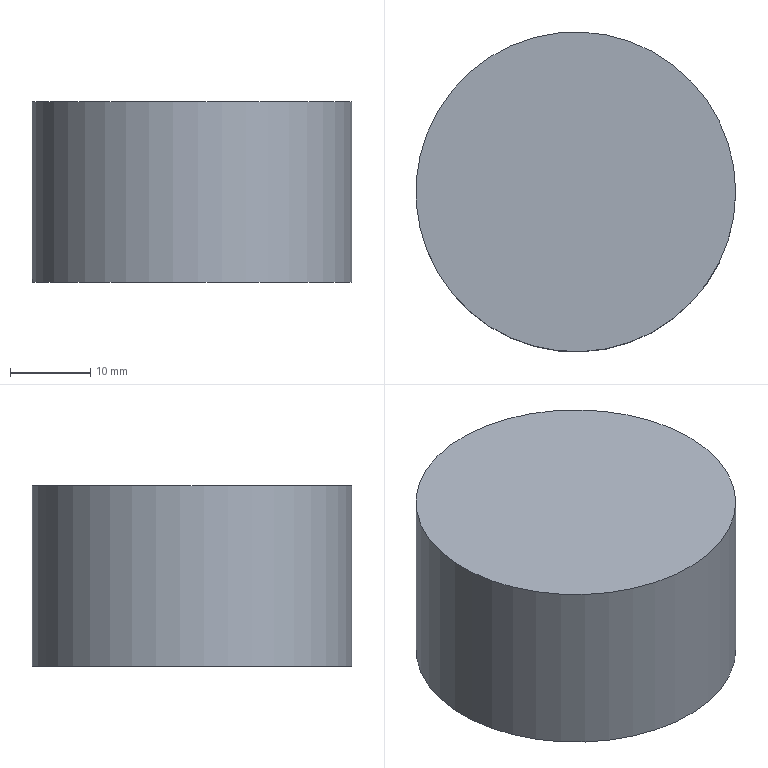Component | NX | SPEAKER | 1 solid | 3 faces | box 39.8 x 39.8 x 22.5 mm | volume 27992 mm3 | plane 2 | cylinder 1 | commonest cylinder face diameters 39.8 x1
STEP:
#1=CARTESIAN_POINT('',(0.,0.,0.));
#2=DIRECTION('',(0.,0.,1.));
#3=DIRECTION('',(1.,0.,0.));
#4=AXIS2_PLACEMENT_3D('',#1,#2,#3);
#5=CARTESIAN_POINT('',(62.178,-1.116,28.276));
#6=VERTEX_POINT('',#5);
#7=CARTESIAN_POINT('',(42.278,-1.116,28.276));
#8=DIRECTION('',(0.,0.,-1.));
#9=DIRECTION('',(1.,0.,0.));
#10=AXIS2_PLACEMENT_3D('',#7,#8,#9);
#11=CIRCLE('',#10,19.9);
#12=CARTESIAN_POINT('',(42.278,-1.116,28.276));
#13=DIRECTION('',(0.,0.,1.));
#14=DIRECTION('',(1.,0.,0.));
#15=AXIS2_PLACEMENT_3D('',#12,#13,#14);
#16=PLANE('',#15);
#17=CARTESIAN_POINT('',(19.9,0.));
#18=CARTESIAN_POINT('',(19.9,-34.468));
#19=CARTESIAN_POINT('',(-9.95,-17.234));
#20=CARTESIAN_POINT('',(-39.8,-0.));
#21=CARTESIAN_POINT('',(-9.95,17.234));
#22=CARTESIAN_POINT('',(19.9,34.468));
#23=CARTESIAN_POINT('',(19.9,0.));
#24=(BOUNDED_CURVE()B_SPLINE_CURVE(2,(#17,#18,#19,#20,#21,#22,#23),.UNSPECIFIED.,.T.,.F.)B_SPLINE_CURVE_WITH_KNOTS((1,2,2,2,2,1),(-2.094,0.,2.094,4.189,6.283,8.378),.UNSPECIFIED.)CURVE()GEOMETRIC_REPRESENTATION_ITEM()RATIONAL_B_SPLINE_CURVE((1.,0.5,1.,0.5,1.,0.5,1.))REPRESENTATION_ITEM(''));
#25=(GEOMETRIC_REPRESENTATION_CONTEXT(2)PARAMETRIC_REPRESENTATION_CONTEXT()REPRESENTATION_CONTEXT('',''));
#26=DEFINITIONAL_REPRESENTATION('',(#24),#25);
#27=PCURVE('',#16,#26);
#28=CARTESIAN_POINT('',(42.278,-1.116,5.776));
#29=DIRECTION('',(0.,0.,1.));
#30=DIRECTION('',(1.,0.,0.));
#31=AXIS2_PLACEMENT_3D('',#28,#29,#30);
#32=CYLINDRICAL_SURFACE('',#31,19.9);
#33=CARTESIAN_POINT('',(6.283,22.5));
#34=DIRECTION('',(-1.,0.));
#35=VECTOR('',#34,1.);
#36=LINE('',#33,#35);
#37=(GEOMETRIC_REPRESENTATION_CONTEXT(2)PARAMETRIC_REPRESENTATION_CONTEXT()REPRESENTATION_CONTEXT('',''));
#38=DEFINITIONAL_REPRESENTATION('',(#36),#37);
#39=PCURVE('',#32,#38);
#40=SURFACE_CURVE('',#11,(#27,#39),.PCURVE_S1.);
#41=EDGE_CURVE('',#6,#6,#40,.T.);
#42=ORIENTED_EDGE('',*,*,#41,.F.);
#43=EDGE_LOOP('',(#42));
#44=FACE_BOUND('',#43,.T.);
#45=ADVANCED_FACE('',(#44),#16,.T.);
#46=CARTESIAN_POINT('',(62.178,-1.116,5.776));
#47=VERTEX_POINT('',#46);
#48=CARTESIAN_POINT('',(42.278,-1.116,5.776));
#49=DIRECTION('',(0.,0.,1.));
#50=DIRECTION('',(1.,0.,0.));
#51=AXIS2_PLACEMENT_3D('',#48,#49,#50);
#52=CIRCLE('',#51,19.9);
#53=CARTESIAN_POINT('',(42.278,-1.116,5.776));
#54=DIRECTION('',(0.,0.,-1.));
#55=DIRECTION('',(-1.,0.,0.));
#56=AXIS2_PLACEMENT_3D('',#53,#54,#55);
#57=PLANE('',#56);
#58=CARTESIAN_POINT('',(-19.9,0.));
#59=CARTESIAN_POINT('',(-19.9,34.468));
#60=CARTESIAN_POINT('',(9.95,17.234));
#61=CARTESIAN_POINT('',(39.8,0.));
#62=CARTESIAN_POINT('',(9.95,-17.234));
#63=CARTESIAN_POINT('',(-19.9,-34.468));
#64=CARTESIAN_POINT('',(-19.9,0.));
#65=(BOUNDED_CURVE()B_SPLINE_CURVE(2,(#58,#59,#60,#61,#62,#63,#64),.UNSPECIFIED.,.T.,.F.)B_SPLINE_CURVE_WITH_KNOTS((1,2,2,2,2,1),(-2.094,0.,2.094,4.189,6.283,8.378),.UNSPECIFIED.)CURVE()GEOMETRIC_REPRESENTATION_ITEM()RATIONAL_B_SPLINE_CURVE((1.,0.5,1.,0.5,1.,0.5,1.))REPRESENTATION_ITEM(''));
#66=(GEOMETRIC_REPRESENTATION_CONTEXT(2)PARAMETRIC_REPRESENTATION_CONTEXT()REPRESENTATION_CONTEXT('',''));
#67=DEFINITIONAL_REPRESENTATION('',(#65),#66);
#68=PCURVE('',#57,#67);
#69=CARTESIAN_POINT('',(0.,0.));
#70=DIRECTION('',(1.,0.));
#71=VECTOR('',#70,1.);
#72=LINE('',#69,#71);
#73=(GEOMETRIC_REPRESENTATION_CONTEXT(2)PARAMETRIC_REPRESENTATION_CONTEXT()REPRESENTATION_CONTEXT('',''));
#74=DEFINITIONAL_REPRESENTATION('',(#72),#73);
#75=PCURVE('',#32,#74);
#76=SURFACE_CURVE('',#52,(#68,#75),.PCURVE_S1.);
#77=EDGE_CURVE('',#47,#47,#76,.T.);
#78=ORIENTED_EDGE('',*,*,#77,.F.);
#79=EDGE_LOOP('',(#78));
#80=FACE_BOUND('',#79,.T.);
#81=ADVANCED_FACE('',(#80),#57,.T.);
#82=ORIENTED_EDGE('',*,*,#41,.T.);
#83=CARTESIAN_POINT('',(62.178,-1.116,5.776));
#84=CARTESIAN_POINT('',(62.178,-1.116,28.276));
#85=B_SPLINE_CURVE_WITH_KNOTS('',1,(#83,#84),.UNSPECIFIED.,.F.,.F.,(2,2),(0.,22.5),.PIECEWISE_BEZIER_KNOTS.);
#86=CARTESIAN_POINT('',(0.,0.));
#87=DIRECTION('',(0.,1.));
#88=VECTOR('',#87,1.);
#89=LINE('',#86,#88);
#90=(GEOMETRIC_REPRESENTATION_CONTEXT(2)PARAMETRIC_REPRESENTATION_CONTEXT()REPRESENTATION_CONTEXT('',''));
#91=DEFINITIONAL_REPRESENTATION('',(#89),#90);
#92=PCURVE('',#32,#91);
#93=CARTESIAN_POINT('',(6.283,0.));
#94=DIRECTION('',(0.,1.));
#95=VECTOR('',#94,1.);
#96=LINE('',#93,#95);
#97=(GEOMETRIC_REPRESENTATION_CONTEXT(2)PARAMETRIC_REPRESENTATION_CONTEXT()REPRESENTATION_CONTEXT('',''));
#98=DEFINITIONAL_REPRESENTATION('',(#96),#97);
#99=PCURVE('',#32,#98);
#100=SEAM_CURVE('',#85,(#92,#99),.PCURVE_S1.);
#101=EDGE_CURVE('',#47,#6,#100,.T.);
#102=ORIENTED_EDGE('',*,*,#101,.F.);
#103=ORIENTED_EDGE('',*,*,#77,.T.);
#104=ORIENTED_EDGE('',*,*,#101,.T.);
#105=EDGE_LOOP('',(#82,#102,#103,#104));
#106=FACE_BOUND('',#105,.T.);
#107=ADVANCED_FACE('',(#106),#32,.T.);
#108=CLOSED_SHELL('',(#45,#81,#107));
#109=MANIFOLD_SOLID_BREP('',#108);
#110=(LENGTH_UNIT()NAMED_UNIT(*)SI_UNIT(.MILLI.,.METRE.));
#111=UNCERTAINTY_MEASURE_WITH_UNIT(LENGTH_MEASURE(0.00001),#110,'','');
#112=(NAMED_UNIT(*)PLANE_ANGLE_UNIT()SI_UNIT($,.RADIAN.));
#113=(NAMED_UNIT(*)SI_UNIT($,.STERADIAN.)SOLID_ANGLE_UNIT());
#114=(GEOMETRIC_REPRESENTATION_CONTEXT(3)GLOBAL_UNCERTAINTY_ASSIGNED_CONTEXT((#111))GLOBAL_UNIT_ASSIGNED_CONTEXT((#110,#112,#113))REPRESENTATION_CONTEXT('',''));
#115=ADVANCED_BREP_SHAPE_REPRESENTATION('',(#4,#109),#114);